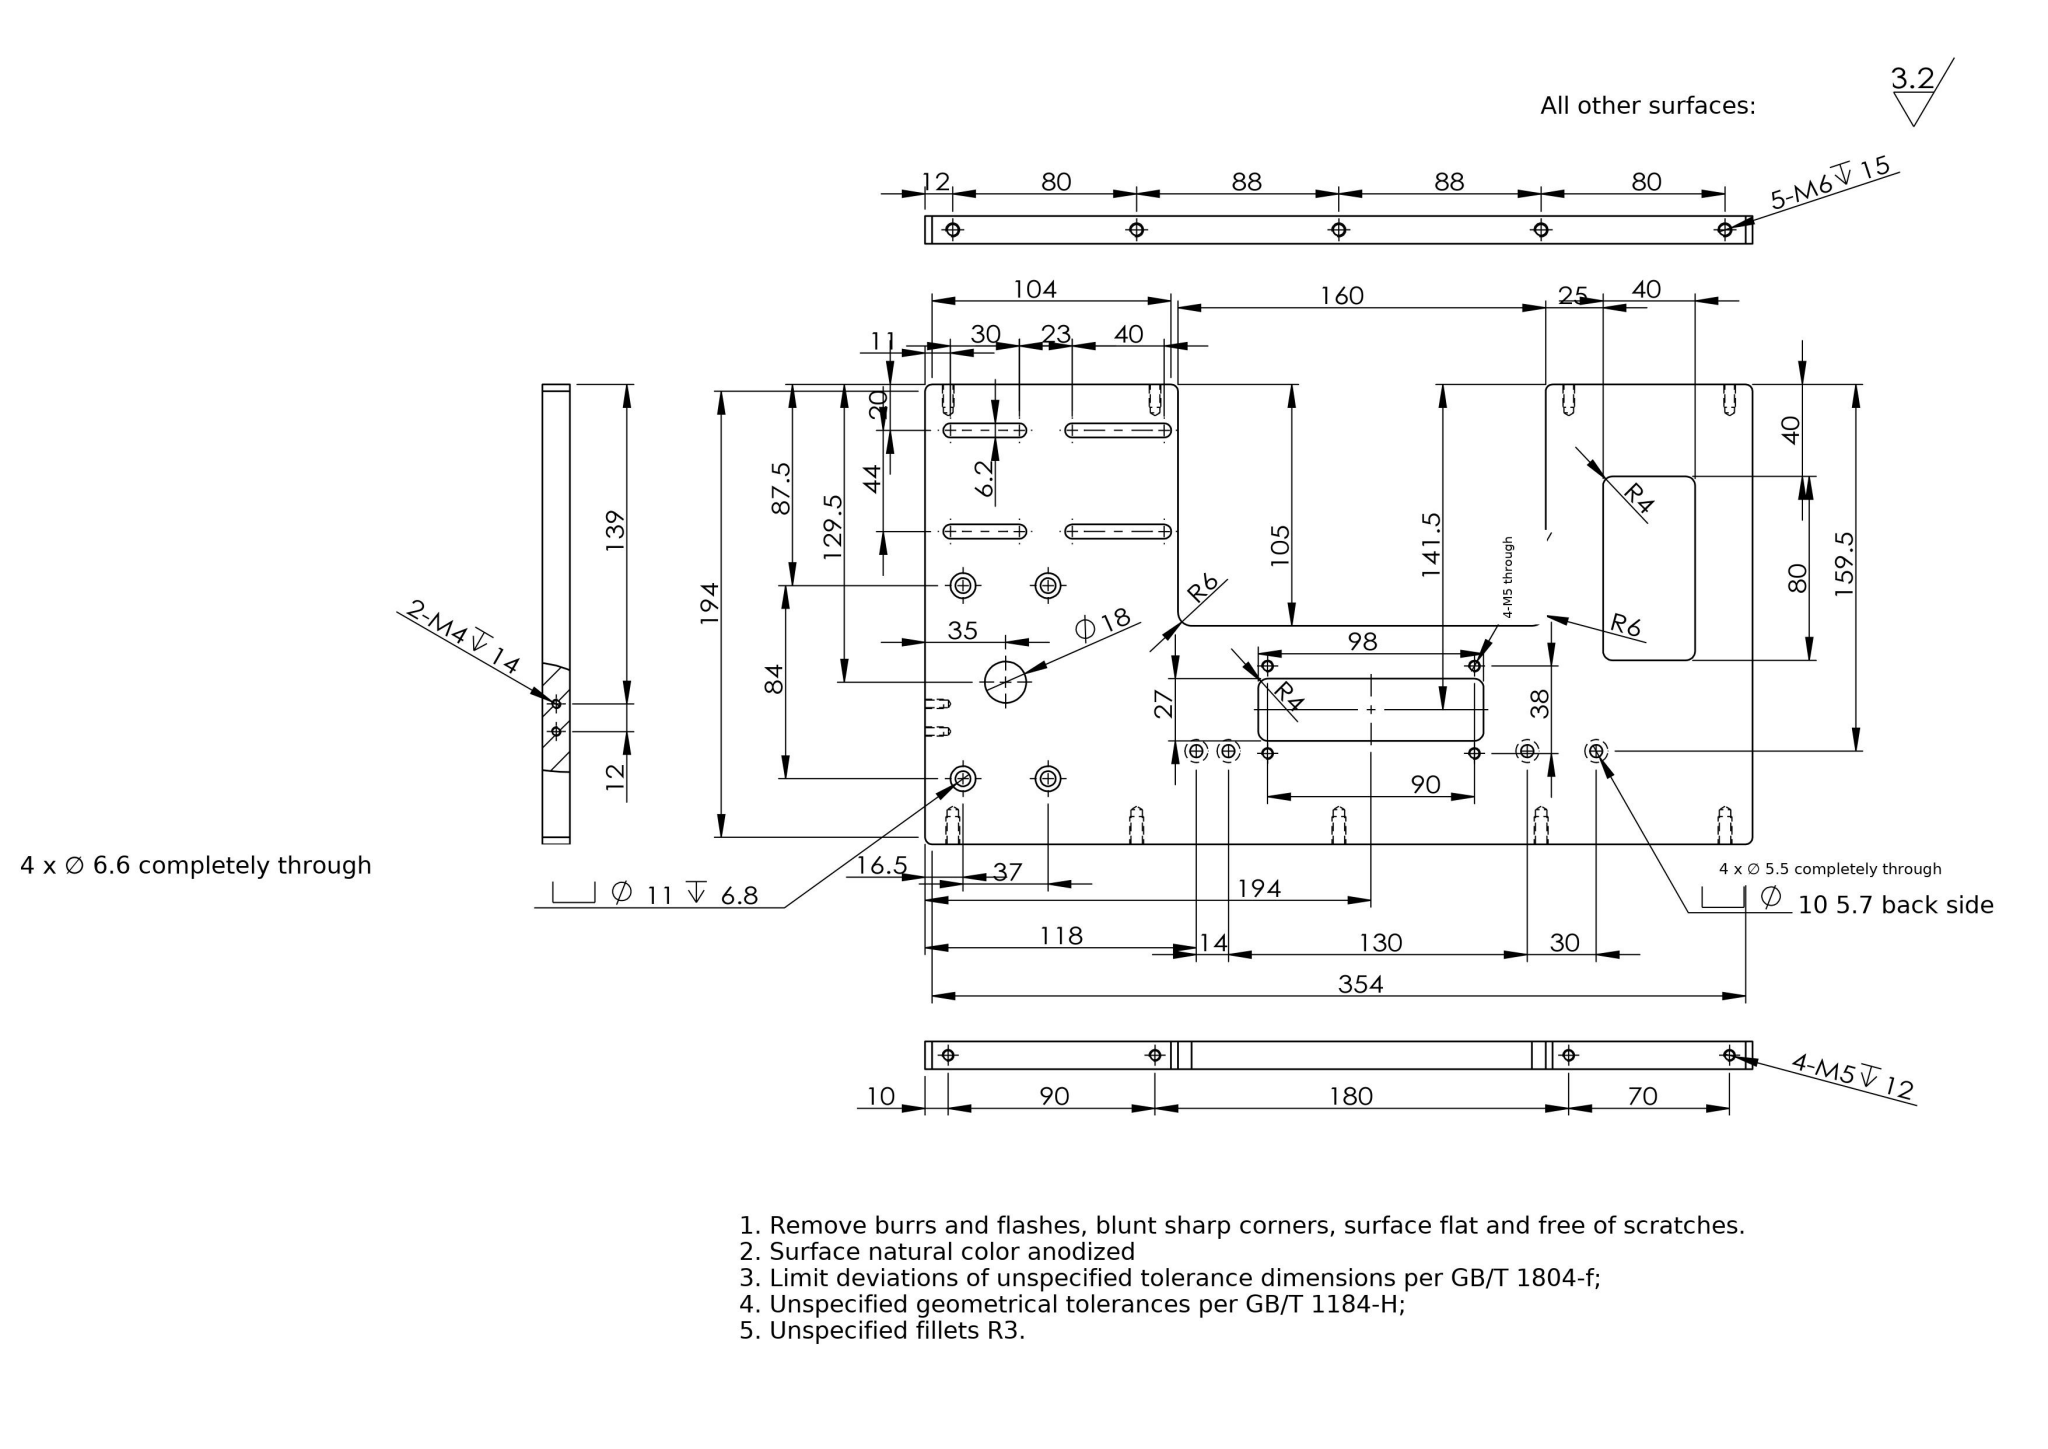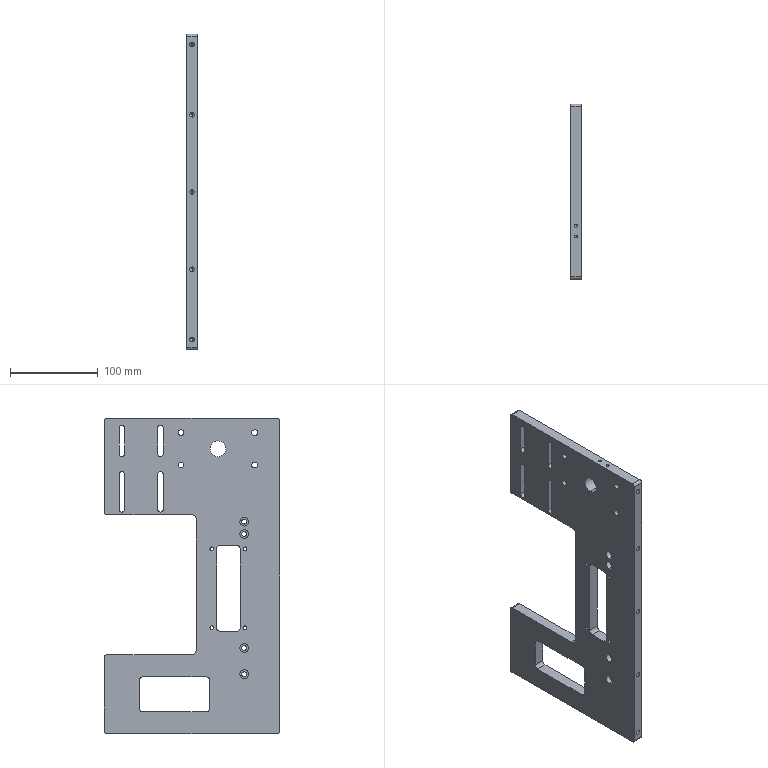Part | SolidWorks | mm | 1 solid | 148 faces | box 12 x 200 x 360 mm | volume 568944 mm3 | cylinder 92 | plane 34 | cone 22 | commonest cylinder face diameters 4.2 x16 6.2 x12 5 x10 10 x8 5.5 x8 11 x8 6.6 x8 8 x8
build123d program:
from build123d import *

# Parameters (mm, degrees)
BOSS_EXTRUDE1_DEPTH                                  = 12
SKETCH2_R                                            = 9
CUT_EXTRUDE1_DEPTH                                   = 57
FILLET1_R                                            = 6
SKETCH3_W                                            = 98
SKETCH3_H                                            = 27
CUT_EXTRUDE2_DEPTH                                   = 30
FILLET2_R                                            = 4
M5_TAPPED_HOLE1_D                                    = 4.2
M5_TAPPED_HOLE1_DEPTH                                = 12.4
M5_TAPPED_HOLE1_TIP                                  = 1.262
CUT_EXTRUDE3_DEPTH                                   = 22
HOLE_SIZE_ACCORDING_TO_TYPE_1_OF_HEXAGON_D           = 6.6
HOLE_SIZE_ACCORDING_TO_TYPE_1_OF_HEXAGON_CBORE_D     = 11
HOLE_SIZE_ACCORDING_TO_TYPE_1_OF_HEXAGON_CBORE_DEPTH = 6.8
M6_TAPPED_HOLE1_D                                    = 5
M6_TAPPED_HOLE1_DEPTH                                = 15
M6_TAPPED_HOLE1_TIP                                  = 1.502
HOLE_SIZE_ACCORDING_TO_TYPE_2_OF_HEXAGON_D           = 5.5
HOLE_SIZE_ACCORDING_TO_TYPE_2_OF_HEXAGON_CBORE_D     = 10
HOLE_SIZE_ACCORDING_TO_TYPE_2_OF_HEXAGON_CBORE_DEPTH = 5.7
M5_TAPPED_HOLE2_D                                    = 4.2
M4_TAPPED_HOLE1_D                                    = 3.3
M4_TAPPED_HOLE1_DEPTH                                = 10.1
M4_TAPPED_HOLE1_TIP                                  = 0.9914
SKETCH17_W                                           = 40
SKETCH17_H                                           = 80
CUT_EXTRUDE4_DEPTH                                   = 31
FILLET3_R                                            = 4
FILLET4_R                                            = 3


with BuildPart() as part:
    # Sketch1 → Boss-Extrude1 (new body)
    with BuildSketch(Plane(origin=(0, 0, 0), x_dir=(0, 0, -1), z_dir=(1, 0, 0))):
        Polygon((0, 0), (0, 200), (110, 200), (110, 95), (270, 95), (270, 200), (360, 200), (360, 0), align=None)
    extrude(amount=BOSS_EXTRUDE1_DEPTH)

    # Sketch2 → Cut-Extrude1 (cut)
    with BuildSketch(Plane.ZY):
        with Locations((-35, 70.5)):
            Circle(SKETCH2_R)
    extrude(amount=-CUT_EXTRUDE1_DEPTH, mode=Mode.SUBTRACT)

    # Fillet1
    fillet1_edges = [part.edges().sort_by_distance(p)[0] for p in [
        (6, 95, -110),
        (6, 95, -270),
    ]]
    fillet(fillet1_edges, radius=FILLET1_R)

    # Sketch3 → Cut-Extrude2 (cut)
    with BuildSketch(Plane(origin=(12, 0, 0), x_dir=(0, 0, -1), z_dir=(1, 0, 0))):
        with Locations((194, 58.5)):
            Rectangle(SKETCH3_W, SKETCH3_H)
    extrude(amount=-CUT_EXTRUDE2_DEPTH, mode=Mode.SUBTRACT)

    # Fillet2
    fillet2_edges = [part.edges().sort_by_distance(p)[0] for p in [
        (6, 45, -145),
        (6, 72, -145),
        (6, 72, -243),
        (6, 45, -243),
    ]]
    fillet(fillet2_edges, radius=FILLET2_R)

    # M5 Tapped Hole1
    with Locations(Plane(origin=(0, 200, 0), x_dir=(1, 0, 0), z_dir=(0, 1, 0))):
        with Locations((6, 10), (6, 350), (6, 280), (6, 100)):
            Hole(M5_TAPPED_HOLE1_D / 2, depth=M5_TAPPED_HOLE1_DEPTH)
            with Locations((0, 0, -(M5_TAPPED_HOLE1_DEPTH + M5_TAPPED_HOLE1_TIP / 2))):  # 118° drill point
                Cone(0, M5_TAPPED_HOLE1_D / 2, M5_TAPPED_HOLE1_TIP, mode=Mode.SUBTRACT)

    # Sketch6 → Cut-Extrude3 (cut)
    with BuildSketch(Plane.ZY):
        with BuildLine():
            Line((-104, 183.1), (-64, 183.1))
            ThreePointArc((-64, 183.1), (-60.9, 180), (-64, 176.9))
            Line((-64, 176.9), (-104, 176.9))
            ThreePointArc((-104, 176.9), (-107.1, 180), (-104, 183.1))
        make_face()
        with BuildLine():
            Line((-41, 183.1), (-11, 183.1))
            ThreePointArc((-11, 183.1), (-7.9, 180), (-11, 176.9))
            Line((-11, 176.9), (-41, 176.9))
            ThreePointArc((-41, 176.9), (-44.1, 180), (-41, 183.1))
        make_face()
        with BuildLine():
            Line((-64, 132.9), (-104, 132.9))
            ThreePointArc((-104, 132.9), (-107.1, 136), (-104, 139.1))
            Line((-104, 139.1), (-64, 139.1))
            ThreePointArc((-64, 139.1), (-60.9, 136), (-64, 132.9))
        make_face()
        with BuildLine():
            Line((-41, 139.1), (-11, 139.1))
            ThreePointArc((-11, 139.1), (-7.9, 136), (-11, 132.9))
            Line((-11, 132.9), (-41, 132.9))
            ThreePointArc((-41, 132.9), (-44.1, 136), (-41, 139.1))
        make_face()
    extrude(amount=-CUT_EXTRUDE3_DEPTH, mode=Mode.SUBTRACT)

    # Hole Size_According to_Type 1 of Hexagon (through all)
    with Locations(Plane(origin=(12, 0, 0), x_dir=(0, 0, -1), z_dir=(1, 0, 0))):
        with Locations((16.5, 112.5), (53.5, 112.5), (53.5, 28.5), (16.5, 28.5)):
            CounterBoreHole(HOLE_SIZE_ACCORDING_TO_TYPE_1_OF_HEXAGON_D / 2, HOLE_SIZE_ACCORDING_TO_TYPE_1_OF_HEXAGON_CBORE_D / 2, HOLE_SIZE_ACCORDING_TO_TYPE_1_OF_HEXAGON_CBORE_DEPTH)

    # M6 Tapped Hole1
    with Locations(Plane(origin=(0, 0, 0), x_dir=(-1, 0, 0), z_dir=(0, -1, 0))):
        with Locations((-6, 348), (-6, 268), (-6, 180), (-6, 92), (-6, 12)):
            Hole(M6_TAPPED_HOLE1_D / 2, depth=M6_TAPPED_HOLE1_DEPTH)
            with Locations((0, 0, -(M6_TAPPED_HOLE1_DEPTH + M6_TAPPED_HOLE1_TIP / 2))):  # 118° drill point
                Cone(0, M6_TAPPED_HOLE1_D / 2, M6_TAPPED_HOLE1_TIP, mode=Mode.SUBTRACT)

    # Hole Size_According to_Type 2 of Hexagon (through all)
    with Locations(Plane.ZY):
        with Locations((-262, 40.5), (-292, 40.5), (-132, 40.5), (-118, 40.5)):
            CounterBoreHole(HOLE_SIZE_ACCORDING_TO_TYPE_2_OF_HEXAGON_D / 2, HOLE_SIZE_ACCORDING_TO_TYPE_2_OF_HEXAGON_CBORE_D / 2, HOLE_SIZE_ACCORDING_TO_TYPE_2_OF_HEXAGON_CBORE_DEPTH)

    # M5 Tapped Hole2 (through all)
    with Locations(Plane.ZY):
        with Locations((-239, 77.5), (-239, 39.5), (-149, 39.5), (-149, 77.5)):
            Hole(M5_TAPPED_HOLE2_D / 2)

    # M4 Tapped Hole1
    with Locations(Plane.XY):
        with Locations((6, 61), (6, 49)):
            Hole(M4_TAPPED_HOLE1_D / 2, depth=M4_TAPPED_HOLE1_DEPTH)
            with Locations((0, 0, -(M4_TAPPED_HOLE1_DEPTH + M4_TAPPED_HOLE1_TIP / 2))):  # 118° drill point
                Cone(0, M4_TAPPED_HOLE1_D / 2, M4_TAPPED_HOLE1_TIP, mode=Mode.SUBTRACT)

    # Sketch17 → Cut-Extrude4 (cut)
    with BuildSketch(Plane(origin=(12, 0, 0), x_dir=(0, 0, -1), z_dir=(1, 0, 0))):
        with Locations((315, 120)):
            Rectangle(SKETCH17_W, SKETCH17_H)
    extrude(amount=-CUT_EXTRUDE4_DEPTH, mode=Mode.SUBTRACT)

    # Fillet3
    fillet3_edges = [part.edges().sort_by_distance(p)[0] for p in [
        (6, 80, -295),
        (6, 160, -295),
        (6, 160, -335),
        (6, 80, -335),
    ]]
    fillet(fillet3_edges, radius=FILLET3_R)

    # Fillet4
    fillet4_edges = [part.edges().sort_by_distance(p)[0] for p in [
        (6, 0, 0),
        (6, 200, 0),
        (6, 200, -110),
        (6, 200, -270),
        (6, 200, -360),
        (6, 0, -360),
    ]]
    fillet(fillet4_edges, radius=FILLET4_R)


solid = part.part